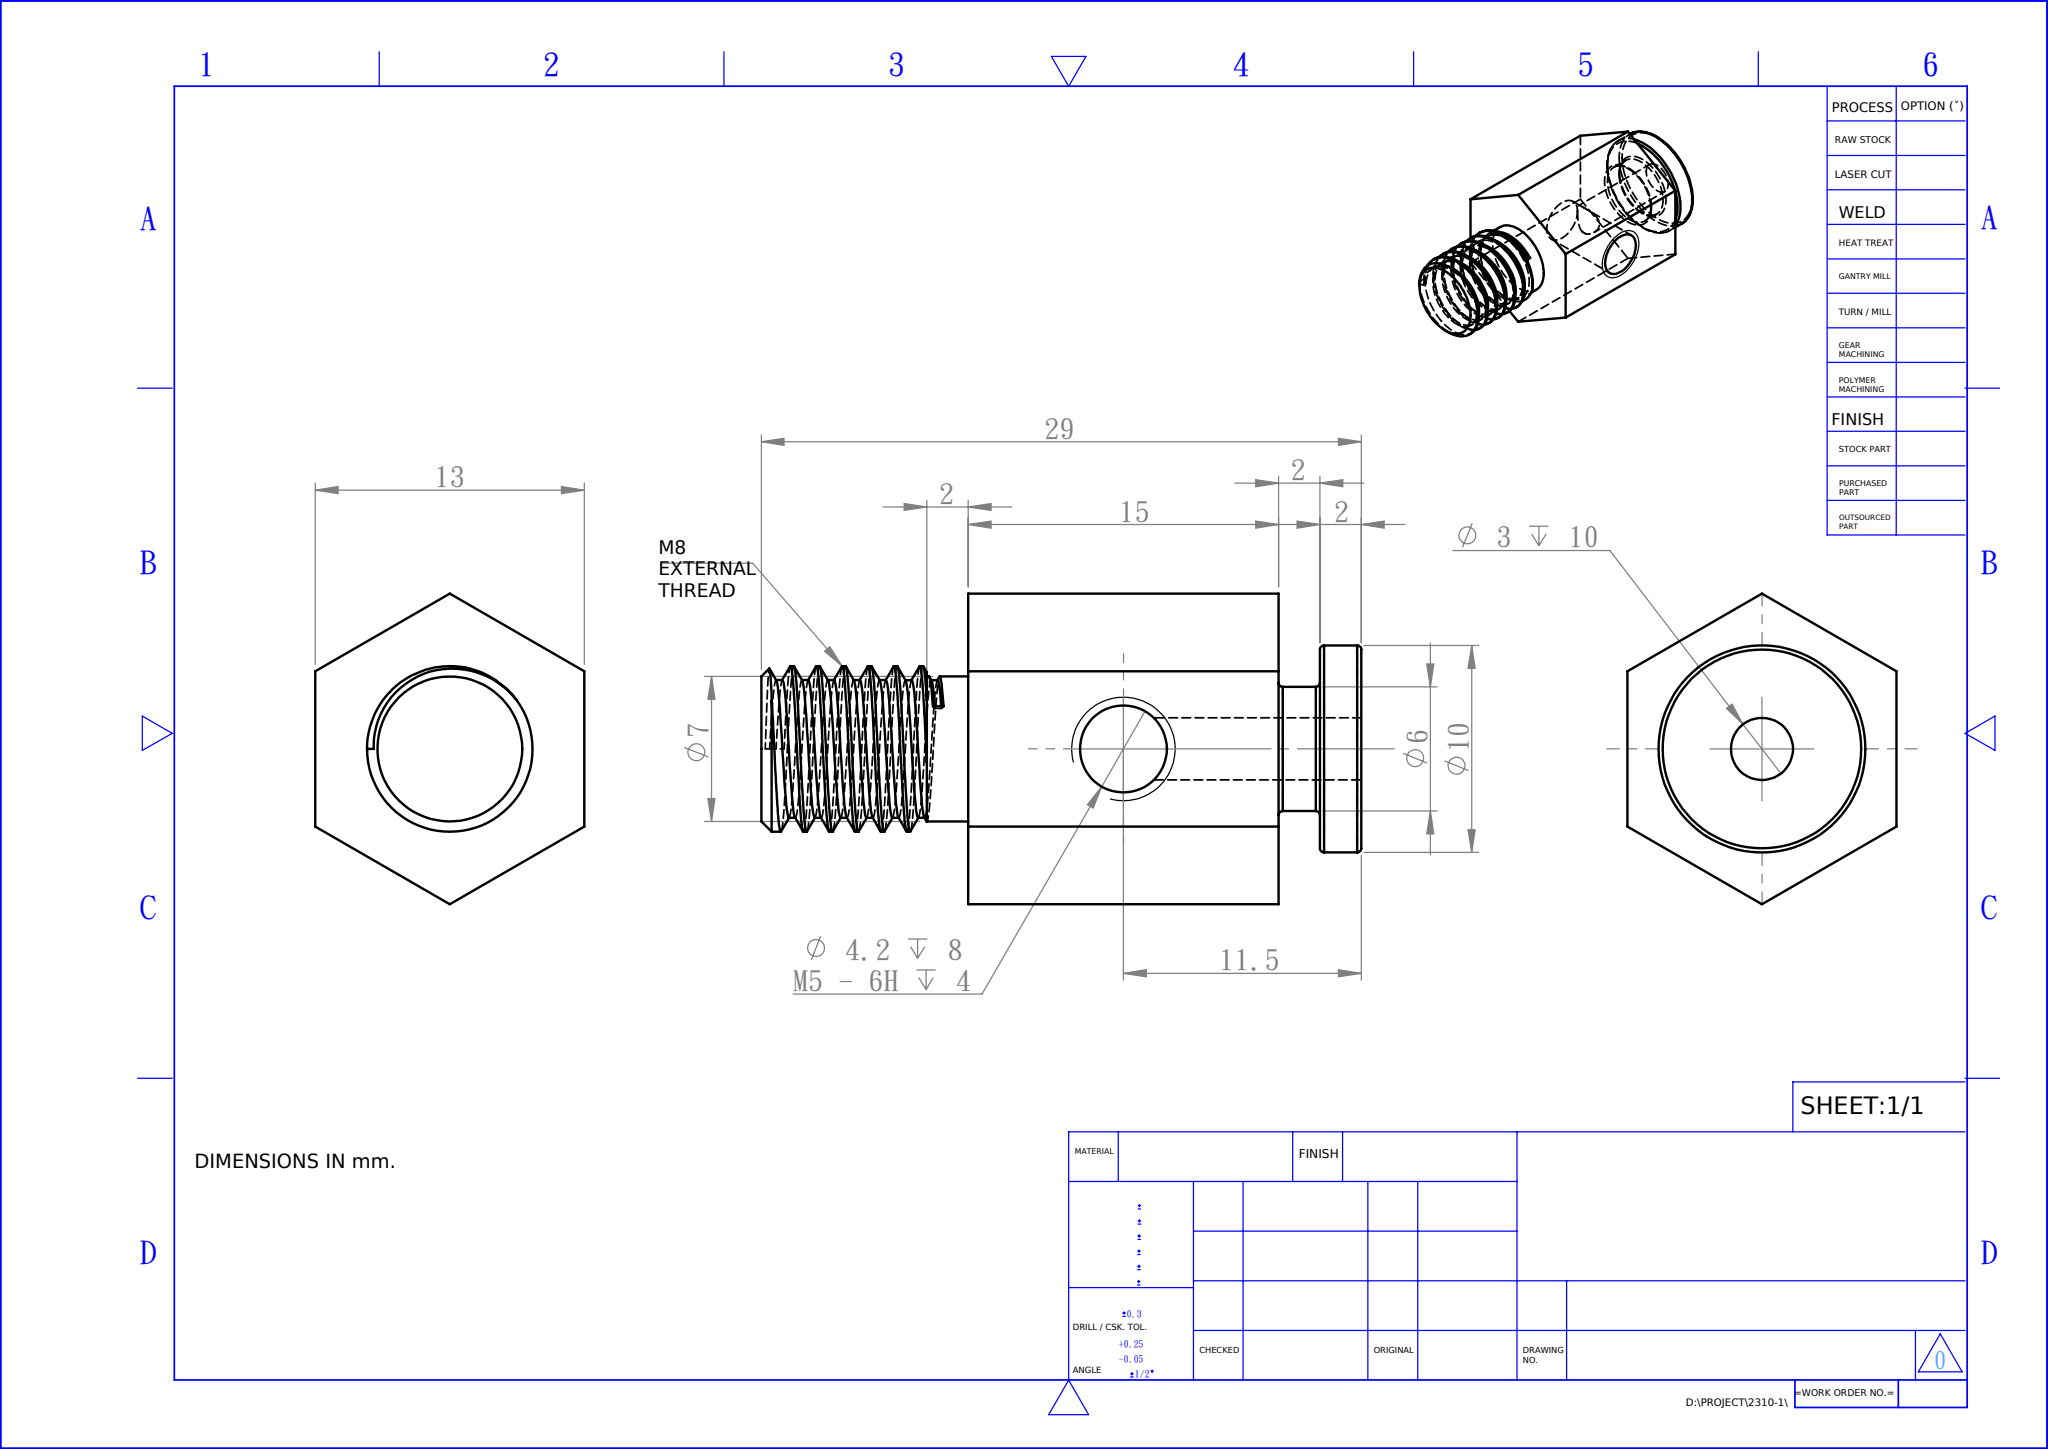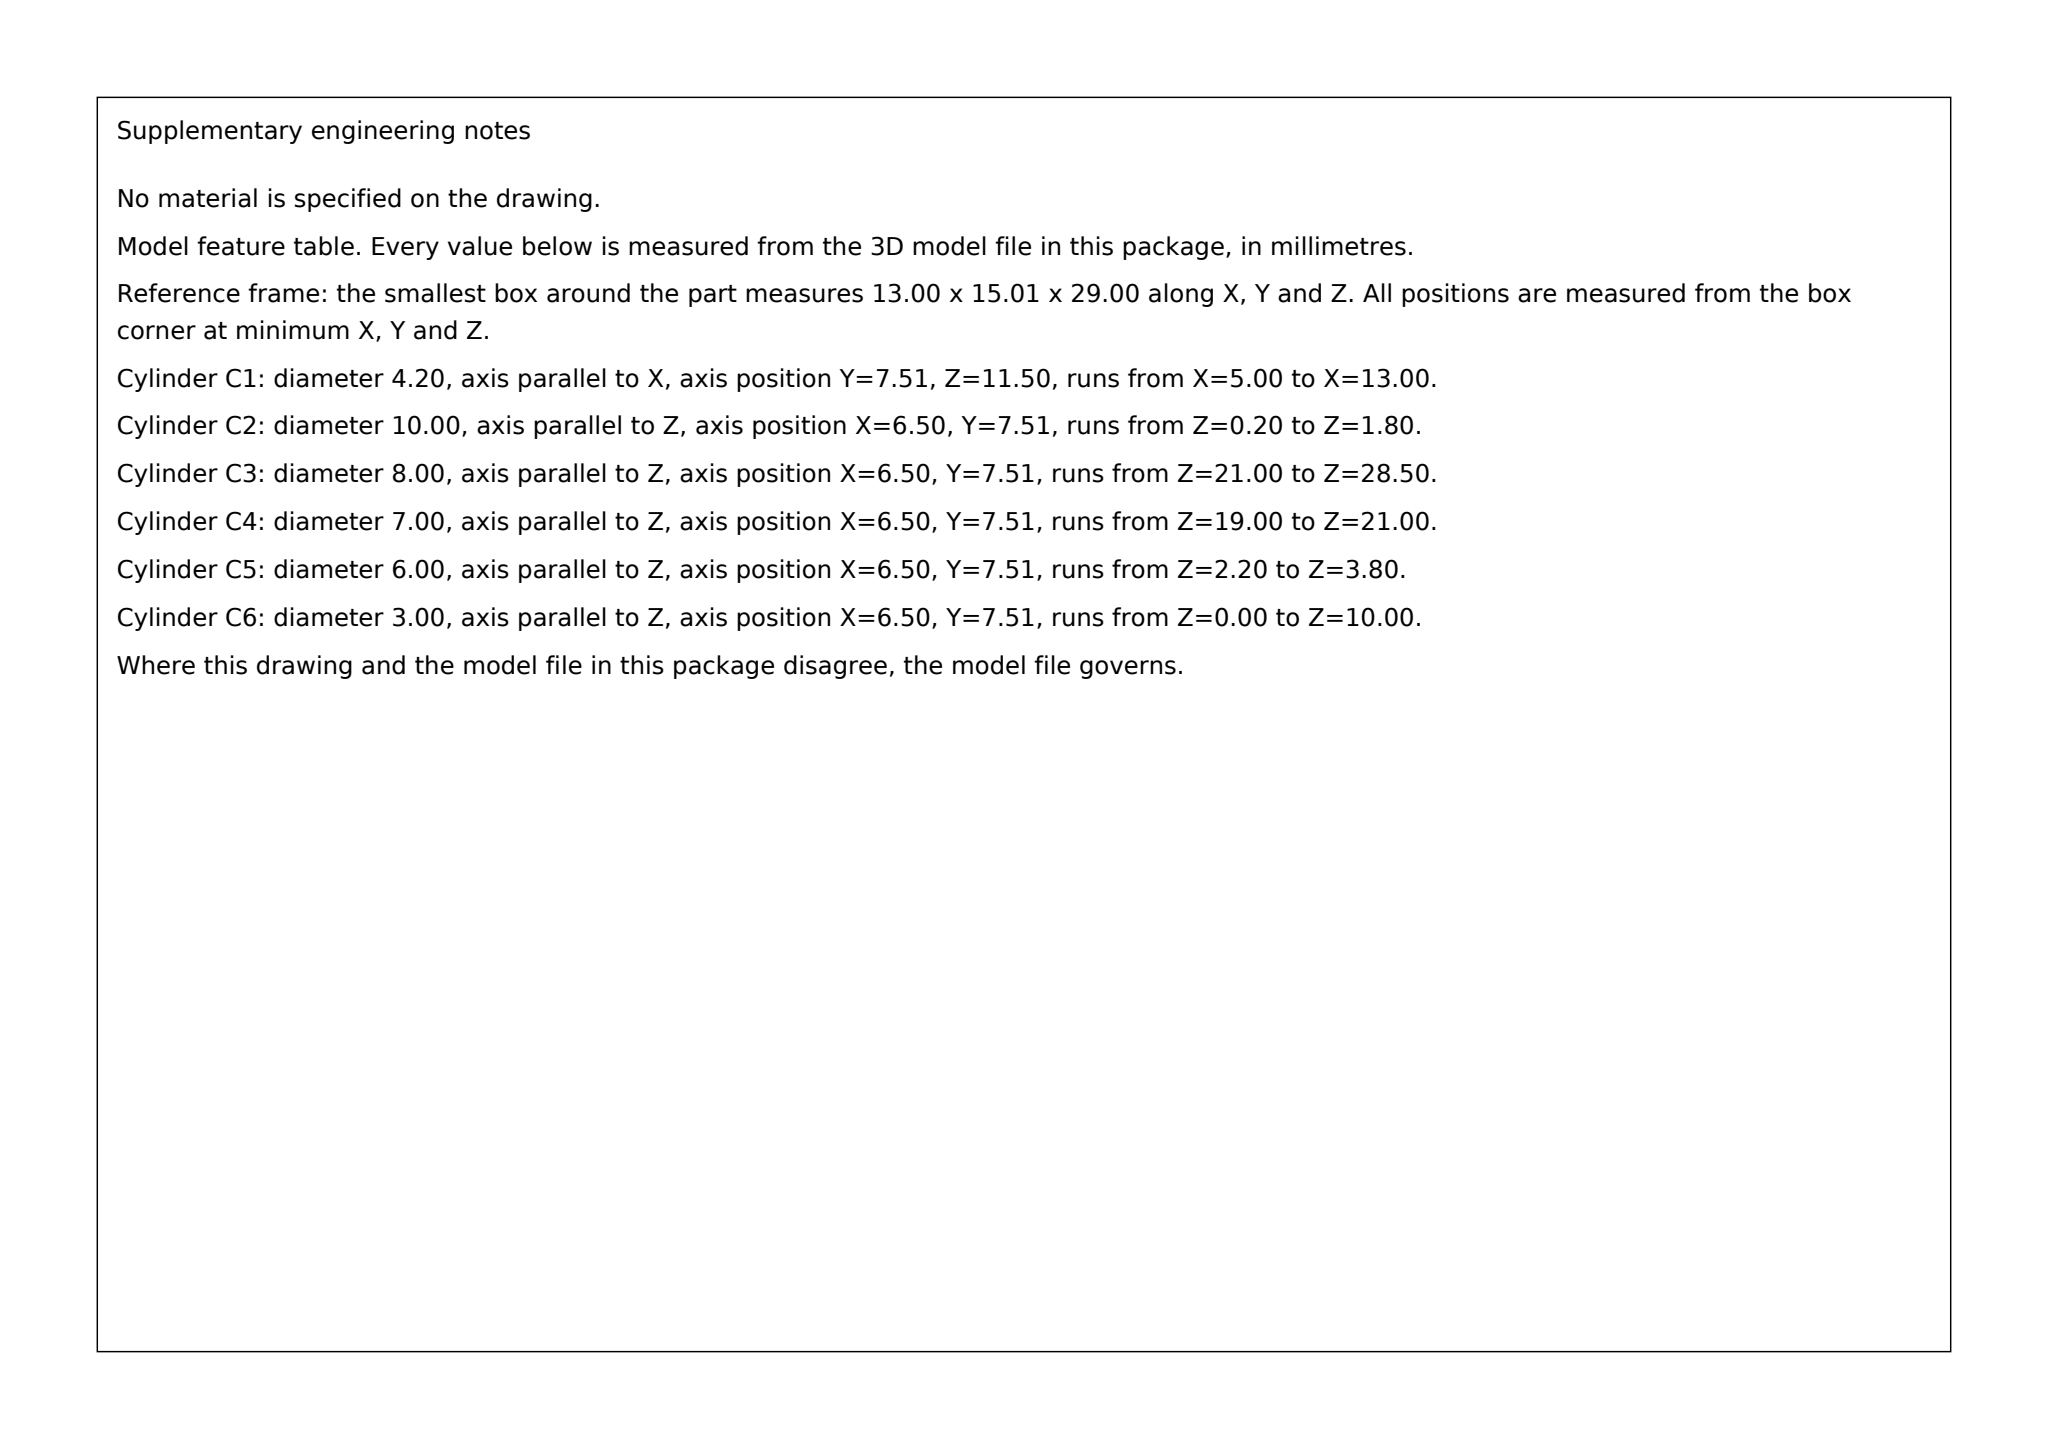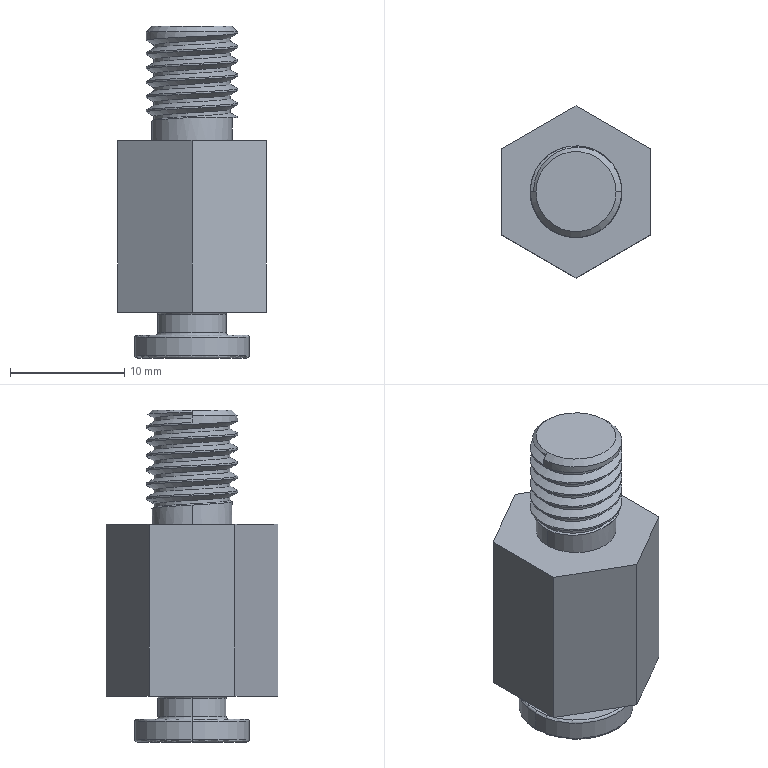Part | SolidWorks | mm | 1 solid | 55 faces | box 13 x 15.01 x 29 mm | volume 2634 mm3 | cylinder 24 | plane 14 | torus 8 | cone 6 | spline 3 | commonest cylinder face diameters 8 x14 4.2 x2 3 x2 10 x2 6 x2 7 x2